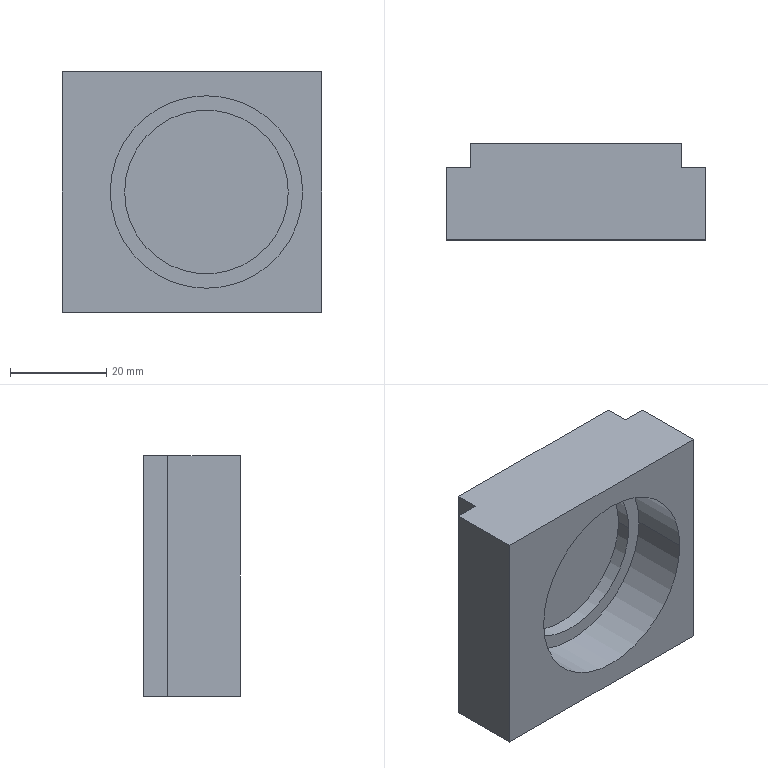Component | SolidWorks | CTM-T-12-AG-04-2 | 1 solid | 16 faces | box 54 x 20 x 50 mm | volume 33697 mm3 | plane 12 | cylinder 4 | commonest cylinder face diameters 34 x2 40 x2 | material Q235A
build123d program:
from build123d import *

# Parameters (mm, degrees)
BOSS_EXTRUDE2_DEPTH = 50
SKETCH3_R           = 20
CUT_EXTRUDE2_DEPTH  = 12
SKETCH7_R           = 17
CUT_EXTRUDE3_DEPTH  = 15


with BuildPart() as part:
    # Sketch1 → Boss-Extrude2 (new body)
    with BuildSketch(Plane.XY):
        Polygon((0, 44), (5, 44), (5, 49), (20, 49), (20, -5), (5, -5), (5, 0), (0, 0), align=None)
    extrude(amount=BOSS_EXTRUDE2_DEPTH)

    # Sketch3 → Cut-Extrude2 (cut)
    with BuildSketch(Plane(origin=(20, 0, 0), x_dir=(0, 0, -1), z_dir=(1, 0, 0))):
        with Locations(Location((-25, 19, 0), (0, 0, 90))):
            Circle(SKETCH3_R)
    extrude(amount=-CUT_EXTRUDE2_DEPTH, mode=Mode.SUBTRACT)

    # Sketch7 → Cut-Extrude3 (cut)
    with BuildSketch(Plane(origin=(20, 0, 0), x_dir=(0, 0, -1), z_dir=(1, 0, 0))):
        with Locations(Location((-25, 19, 0), (0, 0, 90))):
            Circle(SKETCH7_R)
    extrude(amount=-CUT_EXTRUDE3_DEPTH, mode=Mode.SUBTRACT)


solid = part.part

# Placed as in the assembly
solid = solid.moved(Location((59.4, -6, 60), (180, 0, 90)))
STEP:
#1=COLOUR_RGB('',0.7922,0.8196,0.9333);
#2=FILL_AREA_STYLE_COLOUR('',#1);
#3=FILL_AREA_STYLE('',(#2));
#4=SURFACE_STYLE_FILL_AREA(#3);
#5=SURFACE_SIDE_STYLE('',(#4));
#6=SURFACE_STYLE_USAGE(.BOTH.,#5);
#7=PRESENTATION_STYLE_ASSIGNMENT((#6));
#8=CARTESIAN_POINT('',(2.26,-0.4331,1.378));
#9=VERTEX_POINT('',#8);
#10=CARTESIAN_POINT('',(0.9213,-0.4331,1.378));
#11=VERTEX_POINT('',#10);
#12=CARTESIAN_POINT('',(1.591,-0.4331,1.378));
#13=DIRECTION('',(-0.,-1.,-0.));
#14=DIRECTION('',(-1.,0.,0.));
#15=AXIS2_PLACEMENT_3D('',#12,#13,#14);
#16=CIRCLE('',#15,0.6693);
#17=EDGE_CURVE('',#9,#11,#16,.T.);
#18=ORIENTED_EDGE('',*,*,#17,.F.);
#19=CARTESIAN_POINT('',(2.26,-0.5512,1.378));
#20=VERTEX_POINT('',#19);
#21=CARTESIAN_POINT('',(2.26,-0.4331,1.378));
#22=DIRECTION('',(-0.,-1.,-0.));
#23=VECTOR('',#22,39.37);
#24=LINE('',#21,#23);
#25=EDGE_CURVE('',#9,#20,#24,.T.);
#26=ORIENTED_EDGE('',*,*,#25,.T.);
#27=CARTESIAN_POINT('',(0.9213,-0.5512,1.378));
#28=VERTEX_POINT('',#27);
#29=CARTESIAN_POINT('',(1.591,-0.5512,1.378));
#30=DIRECTION('',(-0.,-1.,-0.));
#31=DIRECTION('',(-1.,0.,0.));
#32=AXIS2_PLACEMENT_3D('',#29,#30,#31);
#33=CIRCLE('',#32,0.6693);
#34=EDGE_CURVE('',#20,#28,#33,.T.);
#35=ORIENTED_EDGE('',*,*,#34,.T.);
#36=CARTESIAN_POINT('',(0.9213,-0.4331,1.378));
#37=DIRECTION('',(-0.,-1.,-0.));
#38=VECTOR('',#37,39.37);
#39=LINE('',#36,#38);
#40=EDGE_CURVE('',#11,#28,#39,.T.);
#41=ORIENTED_EDGE('',*,*,#40,.F.);
#42=EDGE_LOOP('',(#18,#26,#35,#41));
#43=FACE_OUTER_BOUND('',#42,.T.);
#44=CARTESIAN_POINT('',(1.591,-0.4331,1.378));
#45=DIRECTION('',(-0.,-1.,-0.));
#46=DIRECTION('',(-1.,0.,0.));
#47=AXIS2_PLACEMENT_3D('',#44,#45,#46);
#48=CYLINDRICAL_SURFACE('',#47,0.6693);
#49=ADVANCED_FACE('',(#43),#48,.F.);
#50=CARTESIAN_POINT('',(2.378,-0.5512,1.378));
#51=VERTEX_POINT('',#50);
#52=CARTESIAN_POINT('',(0.8031,-0.5512,1.378));
#53=VERTEX_POINT('',#52);
#54=CARTESIAN_POINT('',(1.591,-0.5512,1.378));
#55=DIRECTION('',(-0.,-1.,-0.));
#56=DIRECTION('',(-1.,0.,0.));
#57=AXIS2_PLACEMENT_3D('',#54,#55,#56);
#58=CIRCLE('',#57,0.7874);
#59=EDGE_CURVE('',#51,#53,#58,.T.);
#60=ORIENTED_EDGE('',*,*,#59,.F.);
#61=CARTESIAN_POINT('',(2.378,-1.024,1.378));
#62=VERTEX_POINT('',#61);
#63=CARTESIAN_POINT('',(2.378,-0.5512,1.378));
#64=DIRECTION('',(-0.,-1.,-0.));
#65=VECTOR('',#64,39.37);
#66=LINE('',#63,#65);
#67=EDGE_CURVE('',#51,#62,#66,.T.);
#68=ORIENTED_EDGE('',*,*,#67,.T.);
#69=CARTESIAN_POINT('',(0.8031,-1.024,1.378));
#70=VERTEX_POINT('',#69);
#71=CARTESIAN_POINT('',(1.591,-1.024,1.378));
#72=DIRECTION('',(-0.,-1.,-0.));
#73=DIRECTION('',(-1.,0.,0.));
#74=AXIS2_PLACEMENT_3D('',#71,#72,#73);
#75=CIRCLE('',#74,0.7874);
#76=EDGE_CURVE('',#62,#70,#75,.T.);
#77=ORIENTED_EDGE('',*,*,#76,.T.);
#78=CARTESIAN_POINT('',(0.8031,-0.5512,1.378));
#79=DIRECTION('',(-0.,-1.,-0.));
#80=VECTOR('',#79,39.37);
#81=LINE('',#78,#80);
#82=EDGE_CURVE('',#53,#70,#81,.T.);
#83=ORIENTED_EDGE('',*,*,#82,.F.);
#84=EDGE_LOOP('',(#60,#68,#77,#83));
#85=FACE_OUTER_BOUND('',#84,.T.);
#86=CARTESIAN_POINT('',(1.591,-0.5512,1.378));
#87=DIRECTION('',(-0.,-1.,-0.));
#88=DIRECTION('',(-1.,0.,0.));
#89=AXIS2_PLACEMENT_3D('',#86,#87,#88);
#90=CYLINDRICAL_SURFACE('',#89,0.7874);
#91=ADVANCED_FACE('',(#85),#90,.F.);
#92=CARTESIAN_POINT('',(0.6063,-0.2362,2.362));
#93=VERTEX_POINT('',#92);
#94=CARTESIAN_POINT('',(2.339,-0.2362,2.362));
#95=VERTEX_POINT('',#94);
#96=CARTESIAN_POINT('',(2.339,-0.2362,2.362));
#97=DIRECTION('',(1.,-0.,-0.));
#98=VECTOR('',#97,39.37);
#99=LINE('',#96,#98);
#100=EDGE_CURVE('',#93,#95,#99,.T.);
#101=ORIENTED_EDGE('',*,*,#100,.T.);
#102=CARTESIAN_POINT('',(2.339,-0.2362,0.3937));
#103=VERTEX_POINT('',#102);
#104=CARTESIAN_POINT('',(2.339,-0.2362,0.3937));
#105=DIRECTION('',(0.,-0.,1.));
#106=VECTOR('',#105,39.37);
#107=LINE('',#104,#106);
#108=EDGE_CURVE('',#103,#95,#107,.T.);
#109=ORIENTED_EDGE('',*,*,#108,.F.);
#110=CARTESIAN_POINT('',(0.6063,-0.2362,0.3937));
#111=VERTEX_POINT('',#110);
#112=CARTESIAN_POINT('',(2.339,-0.2362,0.3937));
#113=DIRECTION('',(1.,-0.,-0.));
#114=VECTOR('',#113,39.37);
#115=LINE('',#112,#114);
#116=EDGE_CURVE('',#111,#103,#115,.T.);
#117=ORIENTED_EDGE('',*,*,#116,.F.);
#118=CARTESIAN_POINT('',(0.6063,-0.2362,0.3937));
#119=DIRECTION('',(0.,-0.,1.));
#120=VECTOR('',#119,39.37);
#121=LINE('',#118,#120);
#122=EDGE_CURVE('',#111,#93,#121,.T.);
#123=ORIENTED_EDGE('',*,*,#122,.T.);
#124=EDGE_LOOP('',(#101,#109,#117,#123));
#125=FACE_OUTER_BOUND('',#124,.T.);
#126=CARTESIAN_POINT('',(2.339,-0.2362,0.3937));
#127=DIRECTION('',(-0.,-1.,-0.));
#128=DIRECTION('',(0.,-0.,1.));
#129=AXIS2_PLACEMENT_3D('',#126,#127,#128);
#130=PLANE('',#129);
#131=ADVANCED_FACE('',(#125),#130,.F.);
#132=CARTESIAN_POINT('',(2.339,-0.4331,2.362));
#133=VERTEX_POINT('',#132);
#134=CARTESIAN_POINT('',(2.339,-0.4331,2.362));
#135=DIRECTION('',(-0.,-1.,-0.));
#136=VECTOR('',#135,39.37);
#137=LINE('',#134,#136);
#138=EDGE_CURVE('',#95,#133,#137,.T.);
#139=ORIENTED_EDGE('',*,*,#138,.T.);
#140=CARTESIAN_POINT('',(2.339,-0.4331,0.3937));
#141=VERTEX_POINT('',#140);
#142=CARTESIAN_POINT('',(2.339,-0.4331,0.3937));
#143=DIRECTION('',(0.,-0.,1.));
#144=VECTOR('',#143,39.37);
#145=LINE('',#142,#144);
#146=EDGE_CURVE('',#141,#133,#145,.T.);
#147=ORIENTED_EDGE('',*,*,#146,.F.);
#148=CARTESIAN_POINT('',(2.339,-0.4331,0.3937));
#149=DIRECTION('',(-0.,-1.,-0.));
#150=VECTOR('',#149,39.37);
#151=LINE('',#148,#150);
#152=EDGE_CURVE('',#103,#141,#151,.T.);
#153=ORIENTED_EDGE('',*,*,#152,.F.);
#154=ORIENTED_EDGE('',*,*,#108,.T.);
#155=EDGE_LOOP('',(#139,#147,#153,#154));
#156=FACE_OUTER_BOUND('',#155,.T.);
#157=CARTESIAN_POINT('',(2.339,-0.4331,0.3937));
#158=DIRECTION('',(-1.,0.,0.));
#159=DIRECTION('',(0.,1.,0.));
#160=AXIS2_PLACEMENT_3D('',#157,#158,#159);
#161=PLANE('',#160);
#162=ADVANCED_FACE('',(#156),#161,.F.);
#163=CARTESIAN_POINT('',(2.535,-0.4331,2.362));
#164=VERTEX_POINT('',#163);
#165=CARTESIAN_POINT('',(2.535,-0.4331,2.362));
#166=DIRECTION('',(1.,-0.,-0.));
#167=VECTOR('',#166,39.37);
#168=LINE('',#165,#167);
#169=EDGE_CURVE('',#133,#164,#168,.T.);
#170=ORIENTED_EDGE('',*,*,#169,.T.);
#171=CARTESIAN_POINT('',(2.535,-0.4331,0.3937));
#172=VERTEX_POINT('',#171);
#173=CARTESIAN_POINT('',(2.535,-0.4331,0.3937));
#174=DIRECTION('',(0.,-0.,1.));
#175=VECTOR('',#174,39.37);
#176=LINE('',#173,#175);
#177=EDGE_CURVE('',#172,#164,#176,.T.);
#178=ORIENTED_EDGE('',*,*,#177,.F.);
#179=CARTESIAN_POINT('',(2.535,-0.4331,0.3937));
#180=DIRECTION('',(1.,-0.,-0.));
#181=VECTOR('',#180,39.37);
#182=LINE('',#179,#181);
#183=EDGE_CURVE('',#141,#172,#182,.T.);
#184=ORIENTED_EDGE('',*,*,#183,.F.);
#185=ORIENTED_EDGE('',*,*,#146,.T.);
#186=EDGE_LOOP('',(#170,#178,#184,#185));
#187=FACE_OUTER_BOUND('',#186,.T.);
#188=CARTESIAN_POINT('',(2.535,-0.4331,0.3937));
#189=DIRECTION('',(-0.,-1.,-0.));
#190=DIRECTION('',(0.,-0.,1.));
#191=AXIS2_PLACEMENT_3D('',#188,#189,#190);
#192=PLANE('',#191);
#193=ADVANCED_FACE('',(#187),#192,.F.);
#194=CARTESIAN_POINT('',(2.535,-1.024,2.362));
#195=VERTEX_POINT('',#194);
#196=CARTESIAN_POINT('',(2.535,-1.024,2.362));
#197=DIRECTION('',(-0.,-1.,-0.));
#198=VECTOR('',#197,39.37);
#199=LINE('',#196,#198);
#200=EDGE_CURVE('',#164,#195,#199,.T.);
#201=ORIENTED_EDGE('',*,*,#200,.T.);
#202=CARTESIAN_POINT('',(2.535,-1.024,0.3937));
#203=VERTEX_POINT('',#202);
#204=CARTESIAN_POINT('',(2.535,-1.024,0.3937));
#205=DIRECTION('',(0.,-0.,1.));
#206=VECTOR('',#205,39.37);
#207=LINE('',#204,#206);
#208=EDGE_CURVE('',#203,#195,#207,.T.);
#209=ORIENTED_EDGE('',*,*,#208,.F.);
#210=CARTESIAN_POINT('',(2.535,-1.024,0.3937));
#211=DIRECTION('',(-0.,-1.,-0.));
#212=VECTOR('',#211,39.37);
#213=LINE('',#210,#212);
#214=EDGE_CURVE('',#172,#203,#213,.T.);
#215=ORIENTED_EDGE('',*,*,#214,.F.);
#216=ORIENTED_EDGE('',*,*,#177,.T.);
#217=EDGE_LOOP('',(#201,#209,#215,#216));
#218=FACE_OUTER_BOUND('',#217,.T.);
#219=CARTESIAN_POINT('',(2.535,-1.024,0.3937));
#220=DIRECTION('',(-1.,0.,0.));
#221=DIRECTION('',(0.,1.,0.));
#222=AXIS2_PLACEMENT_3D('',#219,#220,#221);
#223=PLANE('',#222);
#224=ADVANCED_FACE('',(#218),#223,.F.);
#225=CARTESIAN_POINT('',(1.591,-1.024,1.378));
#226=DIRECTION('',(-0.,-1.,-0.));
#227=DIRECTION('',(-1.,0.,0.));
#228=AXIS2_PLACEMENT_3D('',#225,#226,#227);
#229=CIRCLE('',#228,0.7874);
#230=EDGE_CURVE('',#70,#62,#229,.T.);
#231=ORIENTED_EDGE('',*,*,#230,.F.);
#232=ORIENTED_EDGE('',*,*,#76,.F.);
#233=EDGE_LOOP('',(#231,#232));
#234=FACE_BOUND('',#233,.T.);
#235=CARTESIAN_POINT('',(0.4094,-1.024,2.362));
#236=VERTEX_POINT('',#235);
#237=CARTESIAN_POINT('',(0.4094,-1.024,2.362));
#238=DIRECTION('',(-1.,0.,0.));
#239=VECTOR('',#238,39.37);
#240=LINE('',#237,#239);
#241=EDGE_CURVE('',#195,#236,#240,.T.);
#242=ORIENTED_EDGE('',*,*,#241,.T.);
#243=CARTESIAN_POINT('',(0.4094,-1.024,0.3937));
#244=VERTEX_POINT('',#243);
#245=CARTESIAN_POINT('',(0.4094,-1.024,0.3937));
#246=DIRECTION('',(0.,-0.,1.));
#247=VECTOR('',#246,39.37);
#248=LINE('',#245,#247);
#249=EDGE_CURVE('',#244,#236,#248,.T.);
#250=ORIENTED_EDGE('',*,*,#249,.F.);
#251=CARTESIAN_POINT('',(0.4094,-1.024,0.3937));
#252=DIRECTION('',(-1.,0.,0.));
#253=VECTOR('',#252,39.37);
#254=LINE('',#251,#253);
#255=EDGE_CURVE('',#203,#244,#254,.T.);
#256=ORIENTED_EDGE('',*,*,#255,.F.);
#257=ORIENTED_EDGE('',*,*,#208,.T.);
#258=EDGE_LOOP('',(#242,#250,#256,#257));
#259=FACE_OUTER_BOUND('',#258,.T.);
#260=CARTESIAN_POINT('',(0.4094,-1.024,0.3937));
#261=DIRECTION('',(0.,1.,0.));
#262=DIRECTION('',(1.,-0.,-0.));
#263=AXIS2_PLACEMENT_3D('',#260,#261,#262);
#264=PLANE('',#263);
#265=ADVANCED_FACE('',(#234,#259),#264,.F.);
#266=CARTESIAN_POINT('',(0.4094,-0.4331,2.362));
#267=VERTEX_POINT('',#266);
#268=CARTESIAN_POINT('',(0.4094,-0.4331,2.362));
#269=DIRECTION('',(0.,1.,0.));
#270=VECTOR('',#269,39.37);
#271=LINE('',#268,#270);
#272=EDGE_CURVE('',#236,#267,#271,.T.);
#273=ORIENTED_EDGE('',*,*,#272,.T.);
#274=CARTESIAN_POINT('',(0.4094,-0.4331,0.3937));
#275=VERTEX_POINT('',#274);
#276=CARTESIAN_POINT('',(0.4094,-0.4331,0.3937));
#277=DIRECTION('',(0.,-0.,1.));
#278=VECTOR('',#277,39.37);
#279=LINE('',#276,#278);
#280=EDGE_CURVE('',#275,#267,#279,.T.);
#281=ORIENTED_EDGE('',*,*,#280,.F.);
#282=CARTESIAN_POINT('',(0.4094,-0.4331,0.3937));
#283=DIRECTION('',(0.,1.,0.));
#284=VECTOR('',#283,39.37);
#285=LINE('',#282,#284);
#286=EDGE_CURVE('',#244,#275,#285,.T.);
#287=ORIENTED_EDGE('',*,*,#286,.F.);
#288=ORIENTED_EDGE('',*,*,#249,.T.);
#289=EDGE_LOOP('',(#273,#281,#287,#288));
#290=FACE_OUTER_BOUND('',#289,.T.);
#291=CARTESIAN_POINT('',(0.4094,-0.4331,0.3937));
#292=DIRECTION('',(1.,-0.,-0.));
#293=DIRECTION('',(0.,-0.,1.));
#294=AXIS2_PLACEMENT_3D('',#291,#292,#293);
#295=PLANE('',#294);
#296=ADVANCED_FACE('',(#290),#295,.F.);
#297=CARTESIAN_POINT('',(0.6063,-0.4331,2.362));
#298=VERTEX_POINT('',#297);
#299=CARTESIAN_POINT('',(0.6063,-0.4331,2.362));
#300=DIRECTION('',(1.,-0.,-0.));
#301=VECTOR('',#300,39.37);
#302=LINE('',#299,#301);
#303=EDGE_CURVE('',#267,#298,#302,.T.);
#304=ORIENTED_EDGE('',*,*,#303,.T.);
#305=CARTESIAN_POINT('',(0.6063,-0.4331,0.3937));
#306=VERTEX_POINT('',#305);
#307=CARTESIAN_POINT('',(0.6063,-0.4331,0.3937));
#308=DIRECTION('',(0.,-0.,1.));
#309=VECTOR('',#308,39.37);
#310=LINE('',#307,#309);
#311=EDGE_CURVE('',#306,#298,#310,.T.);
#312=ORIENTED_EDGE('',*,*,#311,.F.);
#313=CARTESIAN_POINT('',(0.6063,-0.4331,0.3937));
#314=DIRECTION('',(1.,-0.,-0.));
#315=VECTOR('',#314,39.37);
#316=LINE('',#313,#315);
#317=EDGE_CURVE('',#275,#306,#316,.T.);
#318=ORIENTED_EDGE('',*,*,#317,.F.);
#319=ORIENTED_EDGE('',*,*,#280,.T.);
#320=EDGE_LOOP('',(#304,#312,#318,#319));
#321=FACE_OUTER_BOUND('',#320,.T.);
#322=CARTESIAN_POINT('',(0.6063,-0.4331,0.3937));
#323=DIRECTION('',(-0.,-1.,-0.));
#324=DIRECTION('',(-1.,0.,0.));
#325=AXIS2_PLACEMENT_3D('',#322,#323,#324);
#326=PLANE('',#325);
#327=ADVANCED_FACE('',(#321),#326,.F.);
#328=CARTESIAN_POINT('',(0.6063,-0.2362,2.362));
#329=DIRECTION('',(0.,1.,0.));
#330=VECTOR('',#329,39.37);
#331=LINE('',#328,#330);
#332=EDGE_CURVE('',#298,#93,#331,.T.);
#333=ORIENTED_EDGE('',*,*,#332,.T.);
#334=ORIENTED_EDGE('',*,*,#122,.F.);
#335=CARTESIAN_POINT('',(0.6063,-0.2362,0.3937));
#336=DIRECTION('',(0.,1.,0.));
#337=VECTOR('',#336,39.37);
#338=LINE('',#335,#337);
#339=EDGE_CURVE('',#306,#111,#338,.T.);
#340=ORIENTED_EDGE('',*,*,#339,.F.);
#341=ORIENTED_EDGE('',*,*,#311,.T.);
#342=EDGE_LOOP('',(#333,#334,#340,#341));
#343=FACE_OUTER_BOUND('',#342,.T.);
#344=CARTESIAN_POINT('',(0.6063,-0.2362,0.3937));
#345=DIRECTION('',(1.,-0.,-0.));
#346=DIRECTION('',(0.,-0.,1.));
#347=AXIS2_PLACEMENT_3D('',#344,#345,#346);
#348=PLANE('',#347);
#349=ADVANCED_FACE('',(#343),#348,.F.);
#350=ORIENTED_EDGE('',*,*,#116,.T.);
#351=ORIENTED_EDGE('',*,*,#152,.T.);
#352=ORIENTED_EDGE('',*,*,#183,.T.);
#353=ORIENTED_EDGE('',*,*,#214,.T.);
#354=ORIENTED_EDGE('',*,*,#255,.T.);
#355=ORIENTED_EDGE('',*,*,#286,.T.);
#356=ORIENTED_EDGE('',*,*,#317,.T.);
#357=ORIENTED_EDGE('',*,*,#339,.T.);
#358=EDGE_LOOP('',(#350,#351,#352,#353,#354,#355,#356,#357));
#359=FACE_OUTER_BOUND('',#358,.T.);
#360=CARTESIAN_POINT('',(0.6063,-0.2362,0.3937));
#361=DIRECTION('',(0.,-0.,1.));
#362=DIRECTION('',(0.,1.,0.));
#363=AXIS2_PLACEMENT_3D('',#360,#361,#362);
#364=PLANE('',#363);
#365=ADVANCED_FACE('',(#359),#364,.F.);
#366=ORIENTED_EDGE('',*,*,#100,.F.);
#367=ORIENTED_EDGE('',*,*,#332,.F.);
#368=ORIENTED_EDGE('',*,*,#303,.F.);
#369=ORIENTED_EDGE('',*,*,#272,.F.);
#370=ORIENTED_EDGE('',*,*,#241,.F.);
#371=ORIENTED_EDGE('',*,*,#200,.F.);
#372=ORIENTED_EDGE('',*,*,#169,.F.);
#373=ORIENTED_EDGE('',*,*,#138,.F.);
#374=EDGE_LOOP('',(#366,#367,#368,#369,#370,#371,#372,#373));
#375=FACE_OUTER_BOUND('',#374,.T.);
#376=CARTESIAN_POINT('',(0.6063,-0.2362,2.362));
#377=DIRECTION('',(0.,-0.,1.));
#378=DIRECTION('',(0.,1.,0.));
#379=AXIS2_PLACEMENT_3D('',#376,#377,#378);
#380=PLANE('',#379);
#381=ADVANCED_FACE('',(#375),#380,.T.);
#382=ORIENTED_EDGE('',*,*,#67,.F.);
#383=CARTESIAN_POINT('',(1.591,-0.5512,1.378));
#384=DIRECTION('',(-0.,-1.,-0.));
#385=DIRECTION('',(-1.,0.,0.));
#386=AXIS2_PLACEMENT_3D('',#383,#384,#385);
#387=CIRCLE('',#386,0.7874);
#388=EDGE_CURVE('',#53,#51,#387,.T.);
#389=ORIENTED_EDGE('',*,*,#388,.F.);
#390=ORIENTED_EDGE('',*,*,#82,.T.);
#391=ORIENTED_EDGE('',*,*,#230,.T.);
#392=EDGE_LOOP('',(#382,#389,#390,#391));
#393=FACE_OUTER_BOUND('',#392,.T.);
#394=CARTESIAN_POINT('',(1.591,-0.5512,1.378));
#395=DIRECTION('',(-0.,-1.,-0.));
#396=DIRECTION('',(-1.,0.,0.));
#397=AXIS2_PLACEMENT_3D('',#394,#395,#396);
#398=CYLINDRICAL_SURFACE('',#397,0.7874);
#399=ADVANCED_FACE('',(#393),#398,.F.);
#400=CARTESIAN_POINT('',(1.591,-0.5512,1.378));
#401=DIRECTION('',(-0.,-1.,-0.));
#402=DIRECTION('',(-1.,0.,0.));
#403=AXIS2_PLACEMENT_3D('',#400,#401,#402);
#404=CIRCLE('',#403,0.6693);
#405=EDGE_CURVE('',#28,#20,#404,.T.);
#406=ORIENTED_EDGE('',*,*,#405,.F.);
#407=ORIENTED_EDGE('',*,*,#34,.F.);
#408=EDGE_LOOP('',(#406,#407));
#409=FACE_BOUND('',#408,.T.);
#410=ORIENTED_EDGE('',*,*,#388,.T.);
#411=ORIENTED_EDGE('',*,*,#59,.T.);
#412=EDGE_LOOP('',(#410,#411));
#413=FACE_OUTER_BOUND('',#412,.T.);
#414=CARTESIAN_POINT('',(1.591,-0.5512,1.378));
#415=DIRECTION('',(-0.,-1.,-0.));
#416=DIRECTION('',(-1.,0.,0.));
#417=AXIS2_PLACEMENT_3D('',#414,#415,#416);
#418=PLANE('',#417);
#419=ADVANCED_FACE('',(#409,#413),#418,.T.);
#420=ORIENTED_EDGE('',*,*,#25,.F.);
#421=CARTESIAN_POINT('',(1.591,-0.4331,1.378));
#422=DIRECTION('',(-0.,-1.,-0.));
#423=DIRECTION('',(-1.,0.,0.));
#424=AXIS2_PLACEMENT_3D('',#421,#422,#423);
#425=CIRCLE('',#424,0.6693);
#426=EDGE_CURVE('',#11,#9,#425,.T.);
#427=ORIENTED_EDGE('',*,*,#426,.F.);
#428=ORIENTED_EDGE('',*,*,#40,.T.);
#429=ORIENTED_EDGE('',*,*,#405,.T.);
#430=EDGE_LOOP('',(#420,#427,#428,#429));
#431=FACE_OUTER_BOUND('',#430,.T.);
#432=CARTESIAN_POINT('',(1.591,-0.4331,1.378));
#433=DIRECTION('',(-0.,-1.,-0.));
#434=DIRECTION('',(-1.,0.,0.));
#435=AXIS2_PLACEMENT_3D('',#432,#433,#434);
#436=CYLINDRICAL_SURFACE('',#435,0.6693);
#437=ADVANCED_FACE('',(#431),#436,.F.);
#438=ORIENTED_EDGE('',*,*,#426,.T.);
#439=ORIENTED_EDGE('',*,*,#17,.T.);
#440=EDGE_LOOP('',(#438,#439));
#441=FACE_OUTER_BOUND('',#440,.T.);
#442=CARTESIAN_POINT('',(1.591,-0.4331,1.378));
#443=DIRECTION('',(-0.,-1.,-0.));
#444=DIRECTION('',(-1.,0.,0.));
#445=AXIS2_PLACEMENT_3D('',#442,#443,#444);
#446=PLANE('',#445);
#447=ADVANCED_FACE('',(#441),#446,.T.);
#448=CLOSED_SHELL('',(#49,#91,#131,#162,#193,#224,#265,#296,#327,#349,#365,#381,#399,#419,#437,#447));
#449=MANIFOLD_SOLID_BREP('',#448);
#450=STYLED_ITEM('',(#7),#449);
#451=(LENGTH_UNIT()NAMED_UNIT(*)SI_UNIT($,.METRE.));
#452=LENGTH_MEASURE_WITH_UNIT(LENGTH_MEASURE(0.0254),#451);
#453=DIMENSIONAL_EXPONENTS(1.,0.,0.,0.,0.,0.,0.);
#454=(CONVERSION_BASED_UNIT('',#452)LENGTH_UNIT()NAMED_UNIT(#453));
#455=UNCERTAINTY_MEASURE_WITH_UNIT(LENGTH_MEASURE(0.00001),#454,'','');
#456=(NAMED_UNIT(*)PLANE_ANGLE_UNIT()SI_UNIT($,.RADIAN.));
#457=(NAMED_UNIT(*)SI_UNIT($,.STERADIAN.)SOLID_ANGLE_UNIT());
#458=(GEOMETRIC_REPRESENTATION_CONTEXT(3)GLOBAL_UNCERTAINTY_ASSIGNED_CONTEXT((#455))GLOBAL_UNIT_ASSIGNED_CONTEXT((#454,#456,#457))REPRESENTATION_CONTEXT('',''));
#459=MECHANICAL_DESIGN_GEOMETRIC_PRESENTATION_REPRESENTATION('',(#450),#458);
#460=PRESENTATION_LAYER_ASSIGNMENT('','',(#450));
#461=CARTESIAN_POINT('',(0.,0.,0.));
#462=DIRECTION('',(0.,0.,1.));
#463=DIRECTION('',(1.,0.,0.));
#464=AXIS2_PLACEMENT_3D('',#461,#462,#463);
#465=(LENGTH_UNIT()NAMED_UNIT(*)SI_UNIT($,.METRE.));
#466=LENGTH_MEASURE_WITH_UNIT(LENGTH_MEASURE(0.0254),#465);
#467=DIMENSIONAL_EXPONENTS(1.,0.,0.,0.,0.,0.,0.);
#468=(CONVERSION_BASED_UNIT('',#466)LENGTH_UNIT()NAMED_UNIT(#467));
#469=UNCERTAINTY_MEASURE_WITH_UNIT(LENGTH_MEASURE(0.00001),#468,'','');
#470=(NAMED_UNIT(*)PLANE_ANGLE_UNIT()SI_UNIT($,.RADIAN.));
#471=(NAMED_UNIT(*)SI_UNIT($,.STERADIAN.)SOLID_ANGLE_UNIT());
#472=(GEOMETRIC_REPRESENTATION_CONTEXT(3)GLOBAL_UNCERTAINTY_ASSIGNED_CONTEXT((#469))GLOBAL_UNIT_ASSIGNED_CONTEXT((#468,#470,#471))REPRESENTATION_CONTEXT('',''));
#473=ADVANCED_BREP_SHAPE_REPRESENTATION('',(#449,#464),#472);